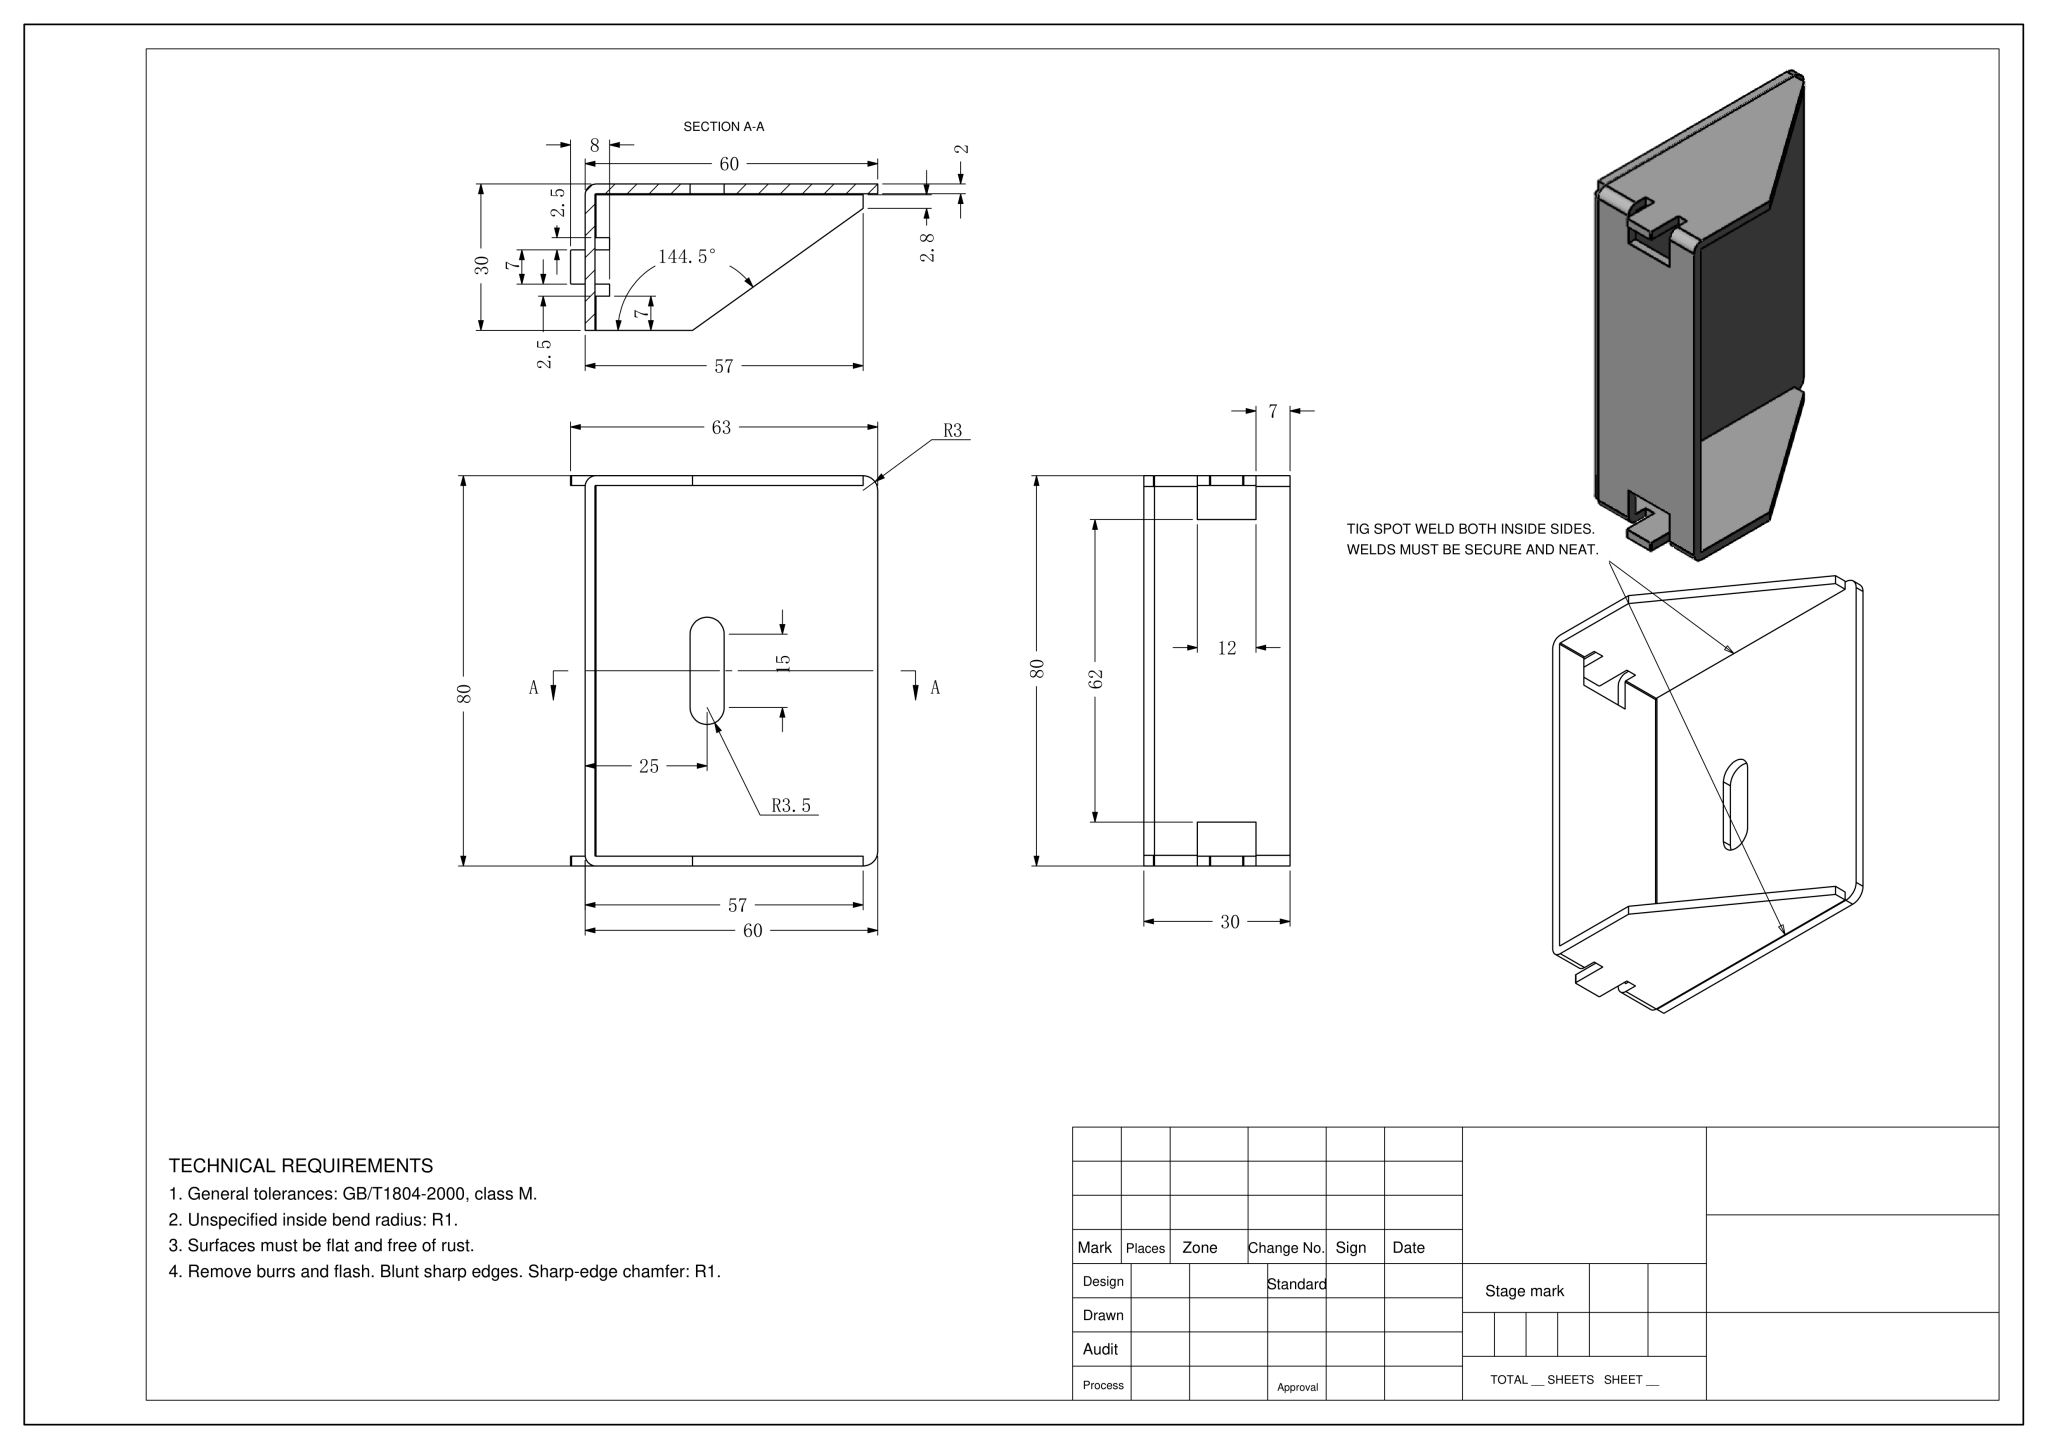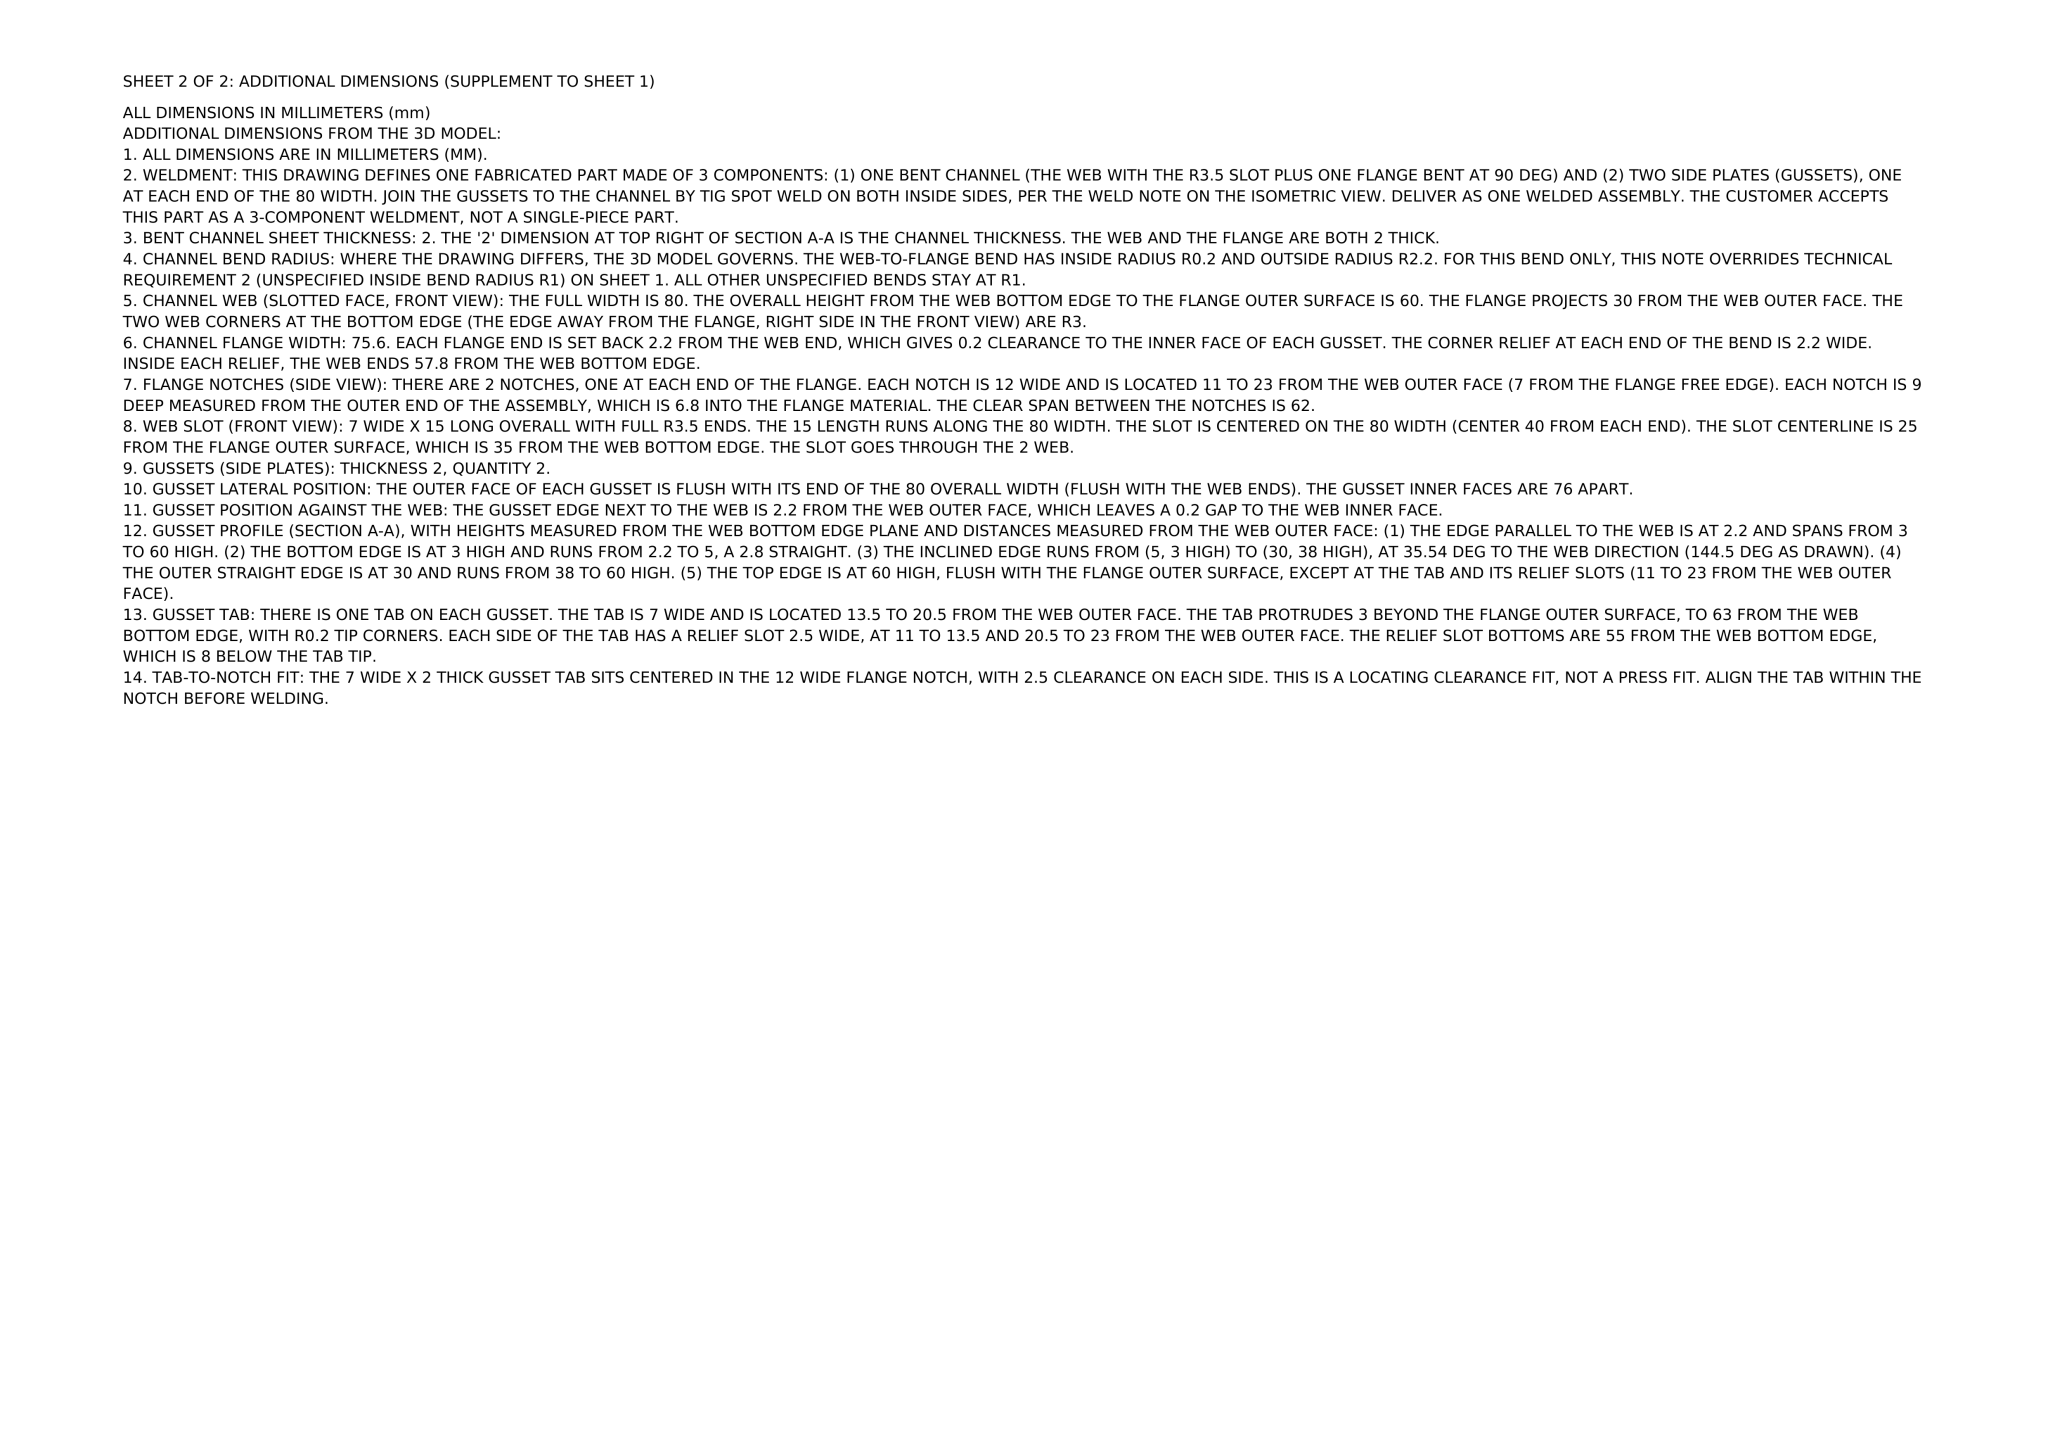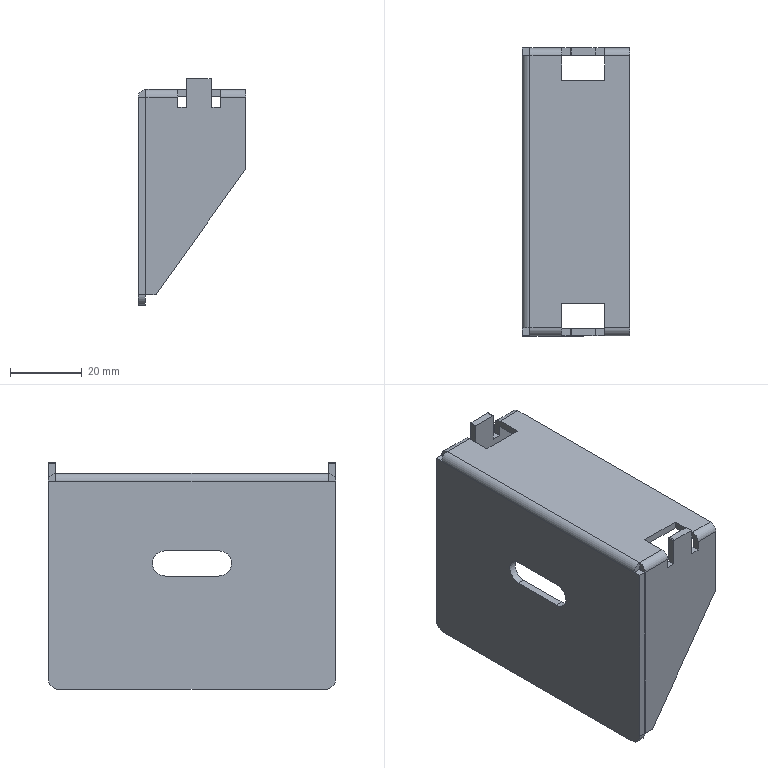Part | NX | mm | Angled Slot Wall Bracket | 1 solid | 58 faces | box 30 x 80 x 63 mm | volume 17668 mm3 | plane 40 | cylinder 18 | commonest cylinder face diameters 0.4 x9 4.4 x5 6 x2 7 x2